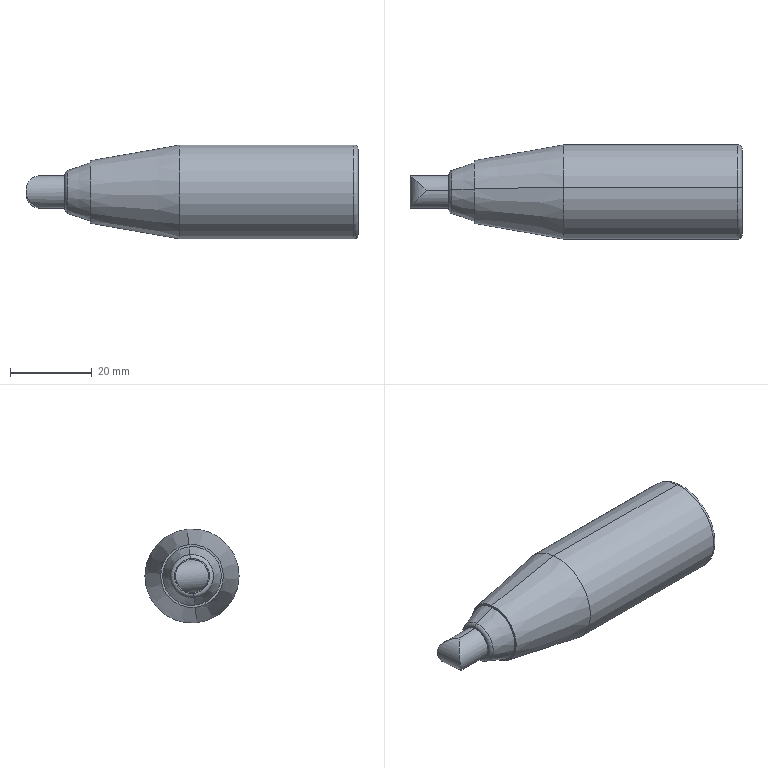Component | SolidWorks | PHSLN125-1_PHSLN_HANDLE125-1 | 1 solid | 16 faces | box 81 x 23 x 23 mm | volume 25609 mm3 | cylinder 5 | torus 4 | cone 4 | plane 3 | commonest cylinder face diameters 8 x3 23 x2
build123d program:
from build123d import *

# Parameters (mm, degrees)
CUT_EXTRUDE1_DEPTH      = 23
CUT_EXTRUDE1_DEPTH_BACK = 23
SKETCH2_W               = 250
SKETCH2_H               = 250


with BuildPart() as part:
    # Sketch1 → Revolve1 (revolve)
    with BuildSketch(Plane.XY, mode=Mode.PRIVATE) as revolve1_sk:
        with BuildLine():
            Line((0, 0), (0, 4))
            Line((0, 4), (9.5, 4))
            Line((9.5, 4), (9.5, 4.29))
            ThreePointArc((9.5, 4.29), (9.685, 4.869), (10.17, 5.234))
            Line((10.17, 5.234), (15.7, 7.167))
            Line((15.7, 7.167), (15.7, 7.667))
            Line((15.7, 7.667), (37.467, 11.5))
            Line((37.467, 11.5), (80, 11.5))
            ThreePointArc((80, 11.5), (80.707, 11.207), (81, 10.5))
            Line((81, 10.5), (81, 0))
            Line((81, 0), (0, 0))
        make_face()
    revolve(revolve1_sk.sketch.rotate(Axis((81, 0, 0), (-1, 0, 0)), 270), axis=Axis((81, 0, 0), (-1, 0, 0)))

    # Sketch2 → Cut-Extrude1 (cut, two sides: drawn at the far end of the back side and taken through both)
    with BuildSketch(Plane(origin=(0, 0, 0), x_dir=(1, 0, 0), z_dir=(0, 1, 0)).offset(-CUT_EXTRUDE1_DEPTH_BACK)):
        with Locations((62.5, 62.5)):
            Rectangle(SKETCH2_W, SKETCH2_H)
        with BuildLine():
            Line((4, -4), (9.5, -4))
            Line((9.5, -4), (9.5, -4.29))
            ThreePointArc((9.5, -4.29), (9.685, -4.869), (10.17, -5.234))
            Line((10.17, -5.234), (15.7, -7.167))
            Line((15.7, -7.167), (15.7, -7.667))
            Line((15.7, -7.667), (37.467, -11.5))
            Line((37.467, -11.5), (80, -11.5))
            ThreePointArc((80, -11.5), (80.707, -11.207), (81, -10.5))
            Line((81, -10.5), (81, 10.5))
            ThreePointArc((81, 10.5), (80.707, 11.207), (80, 11.5))
            Line((80, 11.5), (37.467, 11.5))
            Line((37.467, 11.5), (15.7, 7.667))
            Line((15.7, 7.667), (15.7, 7.167))
            Line((15.7, 7.167), (10.17, 5.234))
            ThreePointArc((10.17, 5.234), (9.685, 4.869), (9.5, 4.29))
            Line((9.5, 4.29), (9.5, 4))
            Line((9.5, 4), (4, 4))
            ThreePointArc((4, 4), (1.172, 2.828), (0, 0))
            ThreePointArc((0, 0), (1.172, -2.828), (4, -4))
        make_face(mode=Mode.SUBTRACT)
    extrude(amount=CUT_EXTRUDE1_DEPTH + CUT_EXTRUDE1_DEPTH_BACK, mode=Mode.SUBTRACT)


solid = part.part

# Placed as in the assembly
solid = solid.moved(Location((601.5, 80.244, -5.079), (174.23, 0, 0)))
STEP:
#1=COLOUR_RGB('',0.7922,0.8196,0.9333);
#2=FILL_AREA_STYLE_COLOUR('',#1);
#3=FILL_AREA_STYLE('',(#2));
#4=SURFACE_STYLE_FILL_AREA(#3);
#5=SURFACE_SIDE_STYLE('',(#4));
#6=SURFACE_STYLE_USAGE(.BOTH.,#5);
#7=PRESENTATION_STYLE_ASSIGNMENT((#6));
#8=CARTESIAN_POINT('',(26.87,3.201,0.2113));
#9=VERTEX_POINT('',#8);
#10=CARTESIAN_POINT('',(26.87,3.118,-0.6112));
#11=VERTEX_POINT('',#10);
#12=CARTESIAN_POINT('',(26.87,3.159,-0.2));
#13=DIRECTION('',(-1.,-0.,0.));
#14=DIRECTION('',(0.,0.1006,0.9949));
#15=AXIS2_PLACEMENT_3D('',#12,#13,#14);
#16=CIRCLE('',#15,0.4134);
#17=EDGE_CURVE('',#9,#11,#16,.T.);
#18=ORIENTED_EDGE('',*,*,#17,.T.);
#19=CARTESIAN_POINT('',(26.831,3.114,-0.6504));
#20=VERTEX_POINT('',#19);
#21=CARTESIAN_POINT('',(26.831,3.118,-0.6112));
#22=DIRECTION('',(-0.,0.9949,-0.1006));
#23=DIRECTION('',(0.,0.1006,0.9949));
#24=AXIS2_PLACEMENT_3D('',#21,#22,#23);
#25=CIRCLE('',#24,0.03937);
#26=EDGE_CURVE('',#11,#20,#25,.T.);
#27=ORIENTED_EDGE('',*,*,#26,.T.);
#28=CARTESIAN_POINT('',(26.831,3.205,0.2505));
#29=VERTEX_POINT('',#28);
#30=CARTESIAN_POINT('',(26.831,3.159,-0.2));
#31=DIRECTION('',(-1.,-0.,0.));
#32=DIRECTION('',(0.,0.1006,0.9949));
#33=AXIS2_PLACEMENT_3D('',#30,#31,#32);
#34=CIRCLE('',#33,0.4528);
#35=EDGE_CURVE('',#29,#20,#34,.T.);
#36=ORIENTED_EDGE('',*,*,#35,.F.);
#37=CARTESIAN_POINT('',(26.831,3.201,0.2113));
#38=DIRECTION('',(0.,-0.9949,0.1006));
#39=DIRECTION('',(0.,-0.1006,-0.9949));
#40=AXIS2_PLACEMENT_3D('',#37,#38,#39);
#41=CIRCLE('',#40,0.03937);
#42=EDGE_CURVE('',#9,#29,#41,.T.);
#43=ORIENTED_EDGE('',*,*,#42,.F.);
#44=EDGE_LOOP('',(#18,#27,#36,#43));
#45=FACE_OUTER_BOUND('',#44,.T.);
#46=CARTESIAN_POINT('',(26.831,3.159,-0.2));
#47=DIRECTION('',(-1.,-0.,0.));
#48=DIRECTION('',(0.,0.1006,0.9949));
#49=AXIS2_PLACEMENT_3D('',#46,#47,#48);
#50=TOROIDAL_SURFACE('',#49,0.4134,0.03937);
#51=ADVANCED_FACE('',(#45),#50,.T.);
#52=ORIENTED_EDGE('',*,*,#35,.T.);
#53=CARTESIAN_POINT('',(25.156,3.114,-0.6504));
#54=VERTEX_POINT('',#53);
#55=CARTESIAN_POINT('',(26.87,3.114,-0.6504));
#56=DIRECTION('',(-1.,-0.,0.));
#57=VECTOR('',#56,39.37);
#58=LINE('',#55,#57);
#59=EDGE_CURVE('',#20,#54,#58,.T.);
#60=ORIENTED_EDGE('',*,*,#59,.T.);
#61=CARTESIAN_POINT('',(25.156,3.205,0.2505));
#62=VERTEX_POINT('',#61);
#63=CARTESIAN_POINT('',(25.156,3.159,-0.2));
#64=DIRECTION('',(-1.,-0.,0.));
#65=DIRECTION('',(0.,0.1006,0.9949));
#66=AXIS2_PLACEMENT_3D('',#63,#64,#65);
#67=CIRCLE('',#66,0.4528);
#68=EDGE_CURVE('',#62,#54,#67,.T.);
#69=ORIENTED_EDGE('',*,*,#68,.F.);
#70=CARTESIAN_POINT('',(26.87,3.205,0.2505));
#71=DIRECTION('',(-1.,-0.,0.));
#72=VECTOR('',#71,39.37);
#73=LINE('',#70,#72);
#74=EDGE_CURVE('',#29,#62,#73,.T.);
#75=ORIENTED_EDGE('',*,*,#74,.F.);
#76=EDGE_LOOP('',(#52,#60,#69,#75));
#77=FACE_OUTER_BOUND('',#76,.T.);
#78=CARTESIAN_POINT('',(26.87,3.159,-0.2));
#79=DIRECTION('',(-1.,-0.,0.));
#80=DIRECTION('',(0.,0.1006,0.9949));
#81=AXIS2_PLACEMENT_3D('',#78,#79,#80);
#82=CYLINDRICAL_SURFACE('',#81,0.4528);
#83=ADVANCED_FACE('',(#77),#82,.T.);
#84=CARTESIAN_POINT('',(24.299,3.19,0.1004));
#85=VERTEX_POINT('',#84);
#86=CARTESIAN_POINT('',(24.299,3.129,-0.5003));
#87=VERTEX_POINT('',#86);
#88=CARTESIAN_POINT('',(24.299,3.159,-0.2));
#89=DIRECTION('',(-1.,-0.,0.));
#90=DIRECTION('',(0.,0.1006,0.9949));
#91=AXIS2_PLACEMENT_3D('',#88,#89,#90);
#92=CIRCLE('',#91,0.3018);
#93=EDGE_CURVE('',#85,#87,#92,.T.);
#94=ORIENTED_EDGE('',*,*,#93,.F.);
#95=CARTESIAN_POINT('',(25.156,3.205,0.2505));
#96=DIRECTION('',(0.9848,0.01744,0.1726));
#97=VECTOR('',#96,39.37);
#98=LINE('',#95,#97);
#99=EDGE_CURVE('',#85,#62,#98,.T.);
#100=ORIENTED_EDGE('',*,*,#99,.T.);
#101=ORIENTED_EDGE('',*,*,#68,.T.);
#102=CARTESIAN_POINT('',(25.156,3.114,-0.6504));
#103=DIRECTION('',(0.9848,-0.01744,-0.1726));
#104=VECTOR('',#103,39.37);
#105=LINE('',#102,#104);
#106=EDGE_CURVE('',#87,#54,#105,.T.);
#107=ORIENTED_EDGE('',*,*,#106,.F.);
#108=EDGE_LOOP('',(#94,#100,#101,#107));
#109=FACE_OUTER_BOUND('',#108,.T.);
#110=CARTESIAN_POINT('',(25.156,3.159,-0.2));
#111=DIRECTION('',(1.,0.,-0.));
#112=DIRECTION('',(0.,-0.1006,-0.9949));
#113=AXIS2_PLACEMENT_3D('',#110,#111,#112);
#114=CONICAL_SURFACE('',#113,0.4528,0.1743);
#115=ADVANCED_FACE('',(#109),#114,.T.);
#116=CARTESIAN_POINT('',(24.082,3.18,0.00507));
#117=VERTEX_POINT('',#116);
#118=CARTESIAN_POINT('',(24.082,3.138,-0.405));
#119=VERTEX_POINT('',#118);
#120=CARTESIAN_POINT('',(24.082,3.159,-0.2));
#121=DIRECTION('',(-1.,-0.,0.));
#122=DIRECTION('',(0.,0.1006,0.9949));
#123=AXIS2_PLACEMENT_3D('',#120,#121,#122);
#124=CIRCLE('',#123,0.2061);
#125=EDGE_CURVE('',#117,#119,#124,.T.);
#126=ORIENTED_EDGE('',*,*,#125,.F.);
#127=CARTESIAN_POINT('',(24.299,3.188,0.08077));
#128=VERTEX_POINT('',#127);
#129=CARTESIAN_POINT('',(24.299,3.188,0.08077));
#130=DIRECTION('',(0.944,0.03318,0.3282));
#131=VECTOR('',#130,39.37);
#132=LINE('',#129,#131);
#133=EDGE_CURVE('',#117,#128,#132,.T.);
#134=ORIENTED_EDGE('',*,*,#133,.T.);
#135=CARTESIAN_POINT('',(24.299,3.131,-0.4807));
#136=VERTEX_POINT('',#135);
#137=CARTESIAN_POINT('',(24.299,3.159,-0.2));
#138=DIRECTION('',(-1.,-0.,0.));
#139=DIRECTION('',(0.,0.1006,0.9949));
#140=AXIS2_PLACEMENT_3D('',#137,#138,#139);
#141=CIRCLE('',#140,0.2822);
#142=EDGE_CURVE('',#128,#136,#141,.T.);
#143=ORIENTED_EDGE('',*,*,#142,.T.);
#144=CARTESIAN_POINT('',(24.299,3.131,-0.4807));
#145=DIRECTION('',(0.944,-0.03318,-0.3282));
#146=VECTOR('',#145,39.37);
#147=LINE('',#144,#146);
#148=EDGE_CURVE('',#119,#136,#147,.T.);
#149=ORIENTED_EDGE('',*,*,#148,.F.);
#150=EDGE_LOOP('',(#126,#134,#143,#149));
#151=FACE_OUTER_BOUND('',#150,.T.);
#152=CARTESIAN_POINT('',(24.299,3.159,-0.2));
#153=DIRECTION('',(1.,0.,-0.));
#154=DIRECTION('',(0.,-0.1006,-0.9949));
#155=AXIS2_PLACEMENT_3D('',#152,#153,#154);
#156=CONICAL_SURFACE('',#155,0.2822,0.3362);
#157=ADVANCED_FACE('',(#151),#156,.T.);
#158=ORIENTED_EDGE('',*,*,#125,.T.);
#159=CARTESIAN_POINT('',(24.055,3.142,-0.368));
#160=VERTEX_POINT('',#159);
#161=CARTESIAN_POINT('',(24.094,3.142,-0.368));
#162=DIRECTION('',(-0.,0.9949,-0.1006));
#163=DIRECTION('',(0.,0.1006,0.9949));
#164=AXIS2_PLACEMENT_3D('',#161,#162,#163);
#165=CIRCLE('',#164,0.03937);
#166=EDGE_CURVE('',#119,#160,#165,.T.);
#167=ORIENTED_EDGE('',*,*,#166,.T.);
#168=CARTESIAN_POINT('',(24.055,3.176,-0.03191));
#169=VERTEX_POINT('',#168);
#170=CARTESIAN_POINT('',(24.055,3.159,-0.2));
#171=DIRECTION('',(-1.,-0.,0.));
#172=DIRECTION('',(0.,0.1006,0.9949));
#173=AXIS2_PLACEMENT_3D('',#170,#171,#172);
#174=CIRCLE('',#173,0.1689);
#175=EDGE_CURVE('',#169,#160,#174,.T.);
#176=ORIENTED_EDGE('',*,*,#175,.F.);
#177=CARTESIAN_POINT('',(24.094,3.176,-0.03191));
#178=DIRECTION('',(0.,-0.9949,0.1006));
#179=DIRECTION('',(0.,-0.1006,-0.9949));
#180=AXIS2_PLACEMENT_3D('',#177,#178,#179);
#181=CIRCLE('',#180,0.03937);
#182=EDGE_CURVE('',#117,#169,#181,.T.);
#183=ORIENTED_EDGE('',*,*,#182,.F.);
#184=EDGE_LOOP('',(#158,#167,#176,#183));
#185=FACE_OUTER_BOUND('',#184,.T.);
#186=CARTESIAN_POINT('',(24.094,3.159,-0.2));
#187=DIRECTION('',(-1.,-0.,0.));
#188=DIRECTION('',(0.,0.1006,0.9949));
#189=AXIS2_PLACEMENT_3D('',#186,#187,#188);
#190=TOROIDAL_SURFACE('',#189,0.1689,0.03937);
#191=ADVANCED_FACE('',(#185),#190,.T.);
#192=CARTESIAN_POINT('',(24.055,3.175,-0.04327));
#193=VERTEX_POINT('',#192);
#194=CARTESIAN_POINT('',(24.055,3.143,-0.3566));
#195=VERTEX_POINT('',#194);
#196=CARTESIAN_POINT('',(24.055,3.159,-0.2));
#197=DIRECTION('',(-1.,-0.,0.));
#198=DIRECTION('',(0.,0.1006,0.9949));
#199=AXIS2_PLACEMENT_3D('',#196,#197,#198);
#200=CIRCLE('',#199,0.1575);
#201=EDGE_CURVE('',#193,#195,#200,.T.);
#202=ORIENTED_EDGE('',*,*,#201,.T.);
#203=CARTESIAN_POINT('',(23.839,3.143,-0.3566));
#204=VERTEX_POINT('',#203);
#205=CARTESIAN_POINT('',(26.87,3.143,-0.3566));
#206=DIRECTION('',(-1.,-0.,0.));
#207=VECTOR('',#206,39.37);
#208=LINE('',#205,#207);
#209=EDGE_CURVE('',#195,#204,#208,.T.);
#210=ORIENTED_EDGE('',*,*,#209,.T.);
#211=CARTESIAN_POINT('',(23.839,3.175,-0.04327));
#212=VERTEX_POINT('',#211);
#213=CARTESIAN_POINT('',(23.839,3.175,-0.04327));
#214=CARTESIAN_POINT('',(23.524,3.488,-0.07495));
#215=CARTESIAN_POINT('',(23.524,3.457,-0.3883));
#216=CARTESIAN_POINT('',(23.839,3.143,-0.3566));
#217=(BOUNDED_CURVE()B_SPLINE_CURVE(3,(#213,#214,#215,#216),.UNSPECIFIED.,.F.,.F.)B_SPLINE_CURVE_WITH_KNOTS((4,4),(4.712,7.854),.UNSPECIFIED.)CURVE()GEOMETRIC_REPRESENTATION_ITEM()RATIONAL_B_SPLINE_CURVE((1.,0.3333,0.3333,1.))REPRESENTATION_ITEM(''));
#218=EDGE_CURVE('',#212,#204,#217,.T.);
#219=ORIENTED_EDGE('',*,*,#218,.F.);
#220=CARTESIAN_POINT('',(26.87,3.175,-0.04327));
#221=DIRECTION('',(-1.,-0.,0.));
#222=VECTOR('',#221,39.37);
#223=LINE('',#220,#222);
#224=EDGE_CURVE('',#193,#212,#223,.T.);
#225=ORIENTED_EDGE('',*,*,#224,.F.);
#226=EDGE_LOOP('',(#202,#210,#219,#225));
#227=FACE_OUTER_BOUND('',#226,.T.);
#228=CARTESIAN_POINT('',(26.87,3.159,-0.2));
#229=DIRECTION('',(-1.,-0.,0.));
#230=DIRECTION('',(0.,0.1006,0.9949));
#231=AXIS2_PLACEMENT_3D('',#228,#229,#230);
#232=CYLINDRICAL_SURFACE('',#231,0.1575);
#233=ADVANCED_FACE('',(#227),#232,.T.);
#234=ORIENTED_EDGE('',*,*,#209,.F.);
#235=CARTESIAN_POINT('',(24.055,3.159,-0.2));
#236=DIRECTION('',(-1.,-0.,0.));
#237=DIRECTION('',(0.,0.1006,0.9949));
#238=AXIS2_PLACEMENT_3D('',#235,#236,#237);
#239=CIRCLE('',#238,0.1575);
#240=EDGE_CURVE('',#195,#193,#239,.T.);
#241=ORIENTED_EDGE('',*,*,#240,.T.);
#242=ORIENTED_EDGE('',*,*,#224,.T.);
#243=CARTESIAN_POINT('',(23.839,3.143,-0.3566));
#244=CARTESIAN_POINT('',(23.524,2.83,-0.325));
#245=CARTESIAN_POINT('',(23.524,2.862,-0.0116));
#246=CARTESIAN_POINT('',(23.839,3.175,-0.04327));
#247=(BOUNDED_CURVE()B_SPLINE_CURVE(3,(#243,#244,#245,#246),.UNSPECIFIED.,.F.,.T.)B_SPLINE_CURVE_WITH_KNOTS((4,4),(4.712,7.854),.UNSPECIFIED.)CURVE()GEOMETRIC_REPRESENTATION_ITEM()RATIONAL_B_SPLINE_CURVE((1.,0.3333,0.3333,1.))REPRESENTATION_ITEM(''));
#248=EDGE_CURVE('',#204,#212,#247,.T.);
#249=ORIENTED_EDGE('',*,*,#248,.F.);
#250=EDGE_LOOP('',(#234,#241,#242,#249));
#251=FACE_OUTER_BOUND('',#250,.T.);
#252=CARTESIAN_POINT('',(26.87,3.159,-0.2));
#253=DIRECTION('',(-1.,-0.,0.));
#254=DIRECTION('',(0.,0.1006,0.9949));
#255=AXIS2_PLACEMENT_3D('',#252,#253,#254);
#256=CYLINDRICAL_SURFACE('',#255,0.1575);
#257=ADVANCED_FACE('',(#251),#256,.T.);
#258=ORIENTED_EDGE('',*,*,#201,.F.);
#259=ORIENTED_EDGE('',*,*,#240,.F.);
#260=EDGE_LOOP('',(#258,#259));
#261=FACE_BOUND('',#260,.T.);
#262=ORIENTED_EDGE('',*,*,#175,.T.);
#263=CARTESIAN_POINT('',(24.055,3.159,-0.2));
#264=DIRECTION('',(-1.,-0.,0.));
#265=DIRECTION('',(0.,0.1006,0.9949));
#266=AXIS2_PLACEMENT_3D('',#263,#264,#265);
#267=CIRCLE('',#266,0.1689);
#268=EDGE_CURVE('',#160,#169,#267,.T.);
#269=ORIENTED_EDGE('',*,*,#268,.T.);
#270=EDGE_LOOP('',(#262,#269));
#271=FACE_OUTER_BOUND('',#270,.T.);
#272=CARTESIAN_POINT('',(24.055,3.316,-0.2158));
#273=DIRECTION('',(1.,0.,-0.));
#274=DIRECTION('',(-0.,-0.1006,-0.9949));
#275=AXIS2_PLACEMENT_3D('',#272,#273,#274);
#276=PLANE('',#275);
#277=ADVANCED_FACE('',(#261,#271),#276,.F.);
#278=ORIENTED_EDGE('',*,*,#166,.F.);
#279=CARTESIAN_POINT('',(24.082,3.159,-0.2));
#280=DIRECTION('',(-1.,-0.,0.));
#281=DIRECTION('',(0.,0.1006,0.9949));
#282=AXIS2_PLACEMENT_3D('',#279,#280,#281);
#283=CIRCLE('',#282,0.2061);
#284=EDGE_CURVE('',#119,#117,#283,.T.);
#285=ORIENTED_EDGE('',*,*,#284,.T.);
#286=ORIENTED_EDGE('',*,*,#182,.T.);
#287=ORIENTED_EDGE('',*,*,#268,.F.);
#288=EDGE_LOOP('',(#278,#285,#286,#287));
#289=FACE_OUTER_BOUND('',#288,.T.);
#290=CARTESIAN_POINT('',(24.094,3.159,-0.2));
#291=DIRECTION('',(-1.,-0.,0.));
#292=DIRECTION('',(0.,0.1006,0.9949));
#293=AXIS2_PLACEMENT_3D('',#290,#291,#292);
#294=TOROIDAL_SURFACE('',#293,0.1689,0.03937);
#295=ADVANCED_FACE('',(#289),#294,.T.);
#296=ORIENTED_EDGE('',*,*,#133,.F.);
#297=ORIENTED_EDGE('',*,*,#284,.F.);
#298=ORIENTED_EDGE('',*,*,#148,.T.);
#299=CARTESIAN_POINT('',(24.299,3.159,-0.2));
#300=DIRECTION('',(-1.,-0.,0.));
#301=DIRECTION('',(0.,0.1006,0.9949));
#302=AXIS2_PLACEMENT_3D('',#299,#300,#301);
#303=CIRCLE('',#302,0.2822);
#304=EDGE_CURVE('',#136,#128,#303,.T.);
#305=ORIENTED_EDGE('',*,*,#304,.T.);
#306=EDGE_LOOP('',(#296,#297,#298,#305));
#307=FACE_OUTER_BOUND('',#306,.T.);
#308=CARTESIAN_POINT('',(24.299,3.159,-0.2));
#309=DIRECTION('',(1.,0.,-0.));
#310=DIRECTION('',(0.,-0.1006,-0.9949));
#311=AXIS2_PLACEMENT_3D('',#308,#309,#310);
#312=CONICAL_SURFACE('',#311,0.2822,0.3362);
#313=ADVANCED_FACE('',(#307),#312,.T.);
#314=ORIENTED_EDGE('',*,*,#304,.F.);
#315=ORIENTED_EDGE('',*,*,#142,.F.);
#316=EDGE_LOOP('',(#314,#315));
#317=FACE_BOUND('',#316,.T.);
#318=CARTESIAN_POINT('',(24.299,3.159,-0.2));
#319=DIRECTION('',(-1.,-0.,0.));
#320=DIRECTION('',(0.,0.1006,0.9949));
#321=AXIS2_PLACEMENT_3D('',#318,#319,#320);
#322=CIRCLE('',#321,0.3018);
#323=EDGE_CURVE('',#87,#85,#322,.T.);
#324=ORIENTED_EDGE('',*,*,#323,.T.);
#325=ORIENTED_EDGE('',*,*,#93,.T.);
#326=EDGE_LOOP('',(#324,#325));
#327=FACE_OUTER_BOUND('',#326,.T.);
#328=CARTESIAN_POINT('',(24.299,3.44,-0.2283));
#329=DIRECTION('',(1.,0.,-0.));
#330=DIRECTION('',(-0.,-0.1006,-0.9949));
#331=AXIS2_PLACEMENT_3D('',#328,#329,#330);
#332=PLANE('',#331);
#333=ADVANCED_FACE('',(#317,#327),#332,.F.);
#334=ORIENTED_EDGE('',*,*,#99,.F.);
#335=ORIENTED_EDGE('',*,*,#323,.F.);
#336=ORIENTED_EDGE('',*,*,#106,.T.);
#337=CARTESIAN_POINT('',(25.156,3.159,-0.2));
#338=DIRECTION('',(-1.,-0.,0.));
#339=DIRECTION('',(0.,0.1006,0.9949));
#340=AXIS2_PLACEMENT_3D('',#337,#338,#339);
#341=CIRCLE('',#340,0.4528);
#342=EDGE_CURVE('',#54,#62,#341,.T.);
#343=ORIENTED_EDGE('',*,*,#342,.T.);
#344=EDGE_LOOP('',(#334,#335,#336,#343));
#345=FACE_OUTER_BOUND('',#344,.T.);
#346=CARTESIAN_POINT('',(25.156,3.159,-0.2));
#347=DIRECTION('',(1.,0.,-0.));
#348=DIRECTION('',(0.,-0.1006,-0.9949));
#349=AXIS2_PLACEMENT_3D('',#346,#347,#348);
#350=CONICAL_SURFACE('',#349,0.4528,0.1743);
#351=ADVANCED_FACE('',(#345),#350,.T.);
#352=ORIENTED_EDGE('',*,*,#59,.F.);
#353=CARTESIAN_POINT('',(26.831,3.159,-0.2));
#354=DIRECTION('',(-1.,-0.,0.));
#355=DIRECTION('',(0.,0.1006,0.9949));
#356=AXIS2_PLACEMENT_3D('',#353,#354,#355);
#357=CIRCLE('',#356,0.4528);
#358=EDGE_CURVE('',#20,#29,#357,.T.);
#359=ORIENTED_EDGE('',*,*,#358,.T.);
#360=ORIENTED_EDGE('',*,*,#74,.T.);
#361=ORIENTED_EDGE('',*,*,#342,.F.);
#362=EDGE_LOOP('',(#352,#359,#360,#361));
#363=FACE_OUTER_BOUND('',#362,.T.);
#364=CARTESIAN_POINT('',(26.87,3.159,-0.2));
#365=DIRECTION('',(-1.,-0.,0.));
#366=DIRECTION('',(0.,0.1006,0.9949));
#367=AXIS2_PLACEMENT_3D('',#364,#365,#366);
#368=CYLINDRICAL_SURFACE('',#367,0.4528);
#369=ADVANCED_FACE('',(#363),#368,.T.);
#370=ORIENTED_EDGE('',*,*,#26,.F.);
#371=CARTESIAN_POINT('',(26.87,3.159,-0.2));
#372=DIRECTION('',(-1.,-0.,0.));
#373=DIRECTION('',(0.,0.1006,0.9949));
#374=AXIS2_PLACEMENT_3D('',#371,#372,#373);
#375=CIRCLE('',#374,0.4134);
#376=EDGE_CURVE('',#11,#9,#375,.T.);
#377=ORIENTED_EDGE('',*,*,#376,.T.);
#378=ORIENTED_EDGE('',*,*,#42,.T.);
#379=ORIENTED_EDGE('',*,*,#358,.F.);
#380=EDGE_LOOP('',(#370,#377,#378,#379));
#381=FACE_OUTER_BOUND('',#380,.T.);
#382=CARTESIAN_POINT('',(26.831,3.159,-0.2));
#383=DIRECTION('',(-1.,-0.,0.));
#384=DIRECTION('',(0.,0.1006,0.9949));
#385=AXIS2_PLACEMENT_3D('',#382,#383,#384);
#386=TOROIDAL_SURFACE('',#385,0.4134,0.03937);
#387=ADVANCED_FACE('',(#381),#386,.T.);
#388=ORIENTED_EDGE('',*,*,#17,.F.);
#389=ORIENTED_EDGE('',*,*,#376,.F.);
#390=EDGE_LOOP('',(#388,#389));
#391=FACE_OUTER_BOUND('',#390,.T.);
#392=CARTESIAN_POINT('',(26.87,3.571,-0.2415));
#393=DIRECTION('',(-1.,-0.,0.));
#394=DIRECTION('',(0.,0.1006,0.9949));
#395=AXIS2_PLACEMENT_3D('',#392,#393,#394);
#396=PLANE('',#395);
#397=ADVANCED_FACE('',(#391),#396,.F.);
#398=ORIENTED_EDGE('',*,*,#218,.T.);
#399=ORIENTED_EDGE('',*,*,#248,.T.);
#400=EDGE_LOOP('',(#398,#399));
#401=FACE_OUTER_BOUND('',#400,.T.);
#402=CARTESIAN_POINT('',(23.839,2.258,-0.1089));
#403=DIRECTION('',(-0.,0.9949,-0.1006));
#404=DIRECTION('',(0.,0.1006,0.9949));
#405=AXIS2_PLACEMENT_3D('',#402,#403,#404);
#406=CYLINDRICAL_SURFACE('',#405,0.1575);
#407=ADVANCED_FACE('',(#401),#406,.T.);
#408=CLOSED_SHELL('',(#51,#83,#115,#157,#191,#233,#257,#277,#295,#313,#333,#351,#369,#387,#397,#407));
#409=MANIFOLD_SOLID_BREP('',#408);
#410=STYLED_ITEM('',(#7),#409);
#411=(LENGTH_UNIT()NAMED_UNIT(*)SI_UNIT($,.METRE.));
#412=LENGTH_MEASURE_WITH_UNIT(LENGTH_MEASURE(0.0254),#411);
#413=DIMENSIONAL_EXPONENTS(1.,0.,0.,0.,0.,0.,0.);
#414=(CONVERSION_BASED_UNIT('',#412)LENGTH_UNIT()NAMED_UNIT(#413));
#415=UNCERTAINTY_MEASURE_WITH_UNIT(LENGTH_MEASURE(0.00001),#414,'','');
#416=(NAMED_UNIT(*)PLANE_ANGLE_UNIT()SI_UNIT($,.RADIAN.));
#417=(NAMED_UNIT(*)SI_UNIT($,.STERADIAN.)SOLID_ANGLE_UNIT());
#418=(GEOMETRIC_REPRESENTATION_CONTEXT(3)GLOBAL_UNCERTAINTY_ASSIGNED_CONTEXT((#415))GLOBAL_UNIT_ASSIGNED_CONTEXT((#414,#416,#417))REPRESENTATION_CONTEXT('',''));
#419=MECHANICAL_DESIGN_GEOMETRIC_PRESENTATION_REPRESENTATION('',(#410),#418);
#420=CARTESIAN_POINT('',(0.,0.,0.));
#421=DIRECTION('',(0.,0.,1.));
#422=DIRECTION('',(1.,0.,0.));
#423=AXIS2_PLACEMENT_3D('',#420,#421,#422);
#424=(LENGTH_UNIT()NAMED_UNIT(*)SI_UNIT($,.METRE.));
#425=LENGTH_MEASURE_WITH_UNIT(LENGTH_MEASURE(0.0254),#424);
#426=DIMENSIONAL_EXPONENTS(1.,0.,0.,0.,0.,0.,0.);
#427=(CONVERSION_BASED_UNIT('',#425)LENGTH_UNIT()NAMED_UNIT(#426));
#428=UNCERTAINTY_MEASURE_WITH_UNIT(LENGTH_MEASURE(0.00001),#427,'','');
#429=(NAMED_UNIT(*)PLANE_ANGLE_UNIT()SI_UNIT($,.RADIAN.));
#430=(NAMED_UNIT(*)SI_UNIT($,.STERADIAN.)SOLID_ANGLE_UNIT());
#431=(GEOMETRIC_REPRESENTATION_CONTEXT(3)GLOBAL_UNCERTAINTY_ASSIGNED_CONTEXT((#428))GLOBAL_UNIT_ASSIGNED_CONTEXT((#427,#429,#430))REPRESENTATION_CONTEXT('',''));
#432=ADVANCED_BREP_SHAPE_REPRESENTATION('',(#409,#423),#431);
#433=PRESENTATION_LAYER_ASSIGNMENT('','',(#410));